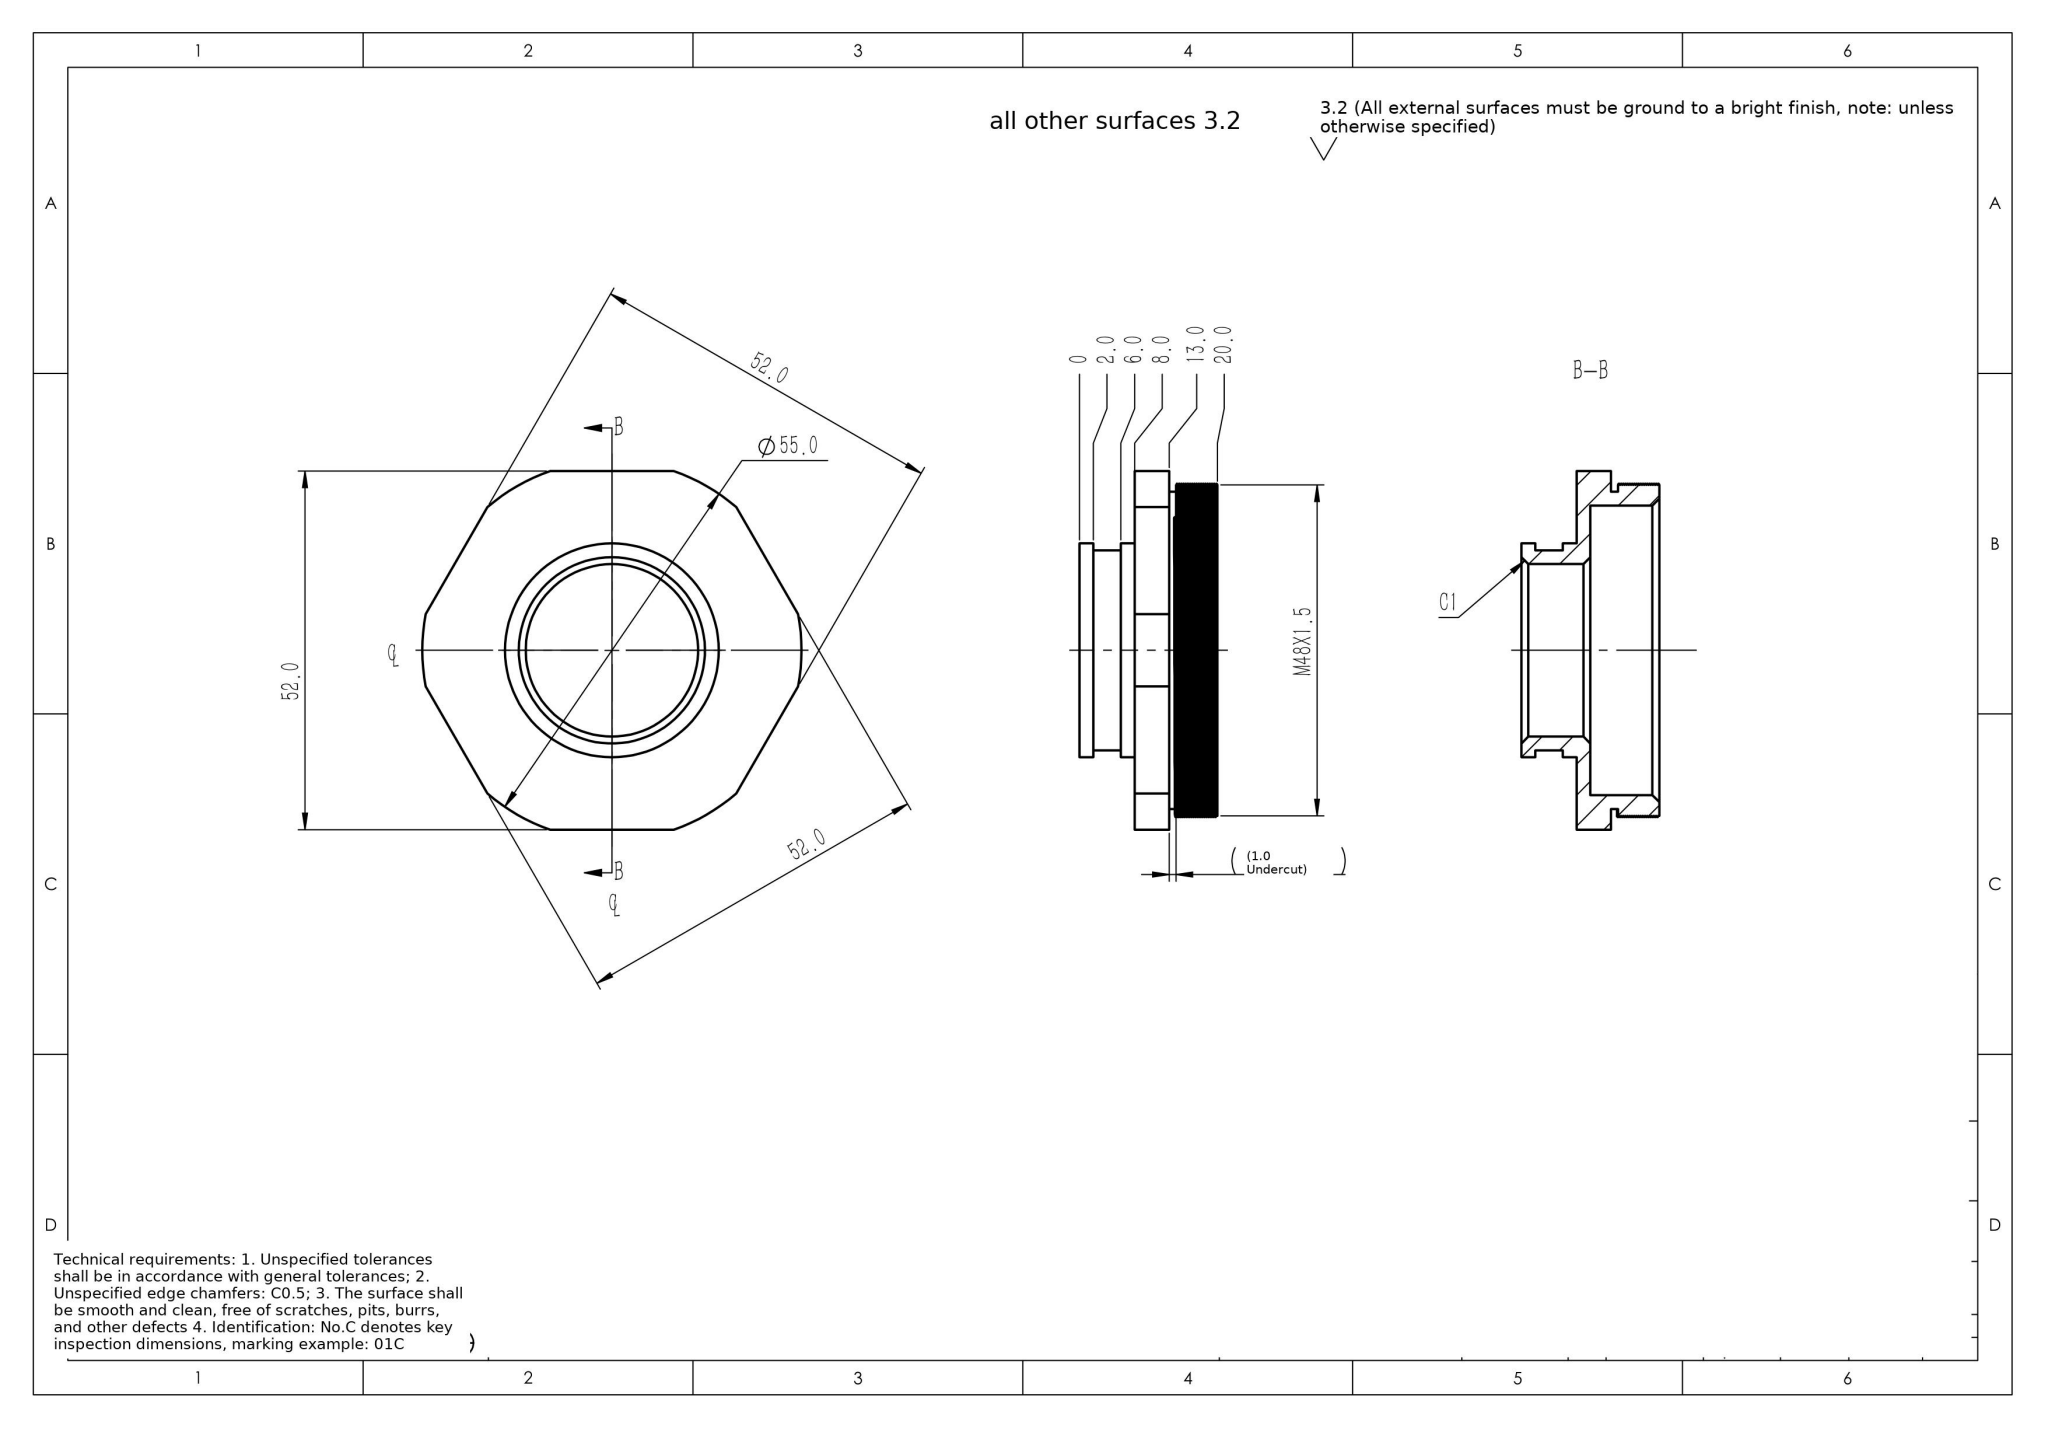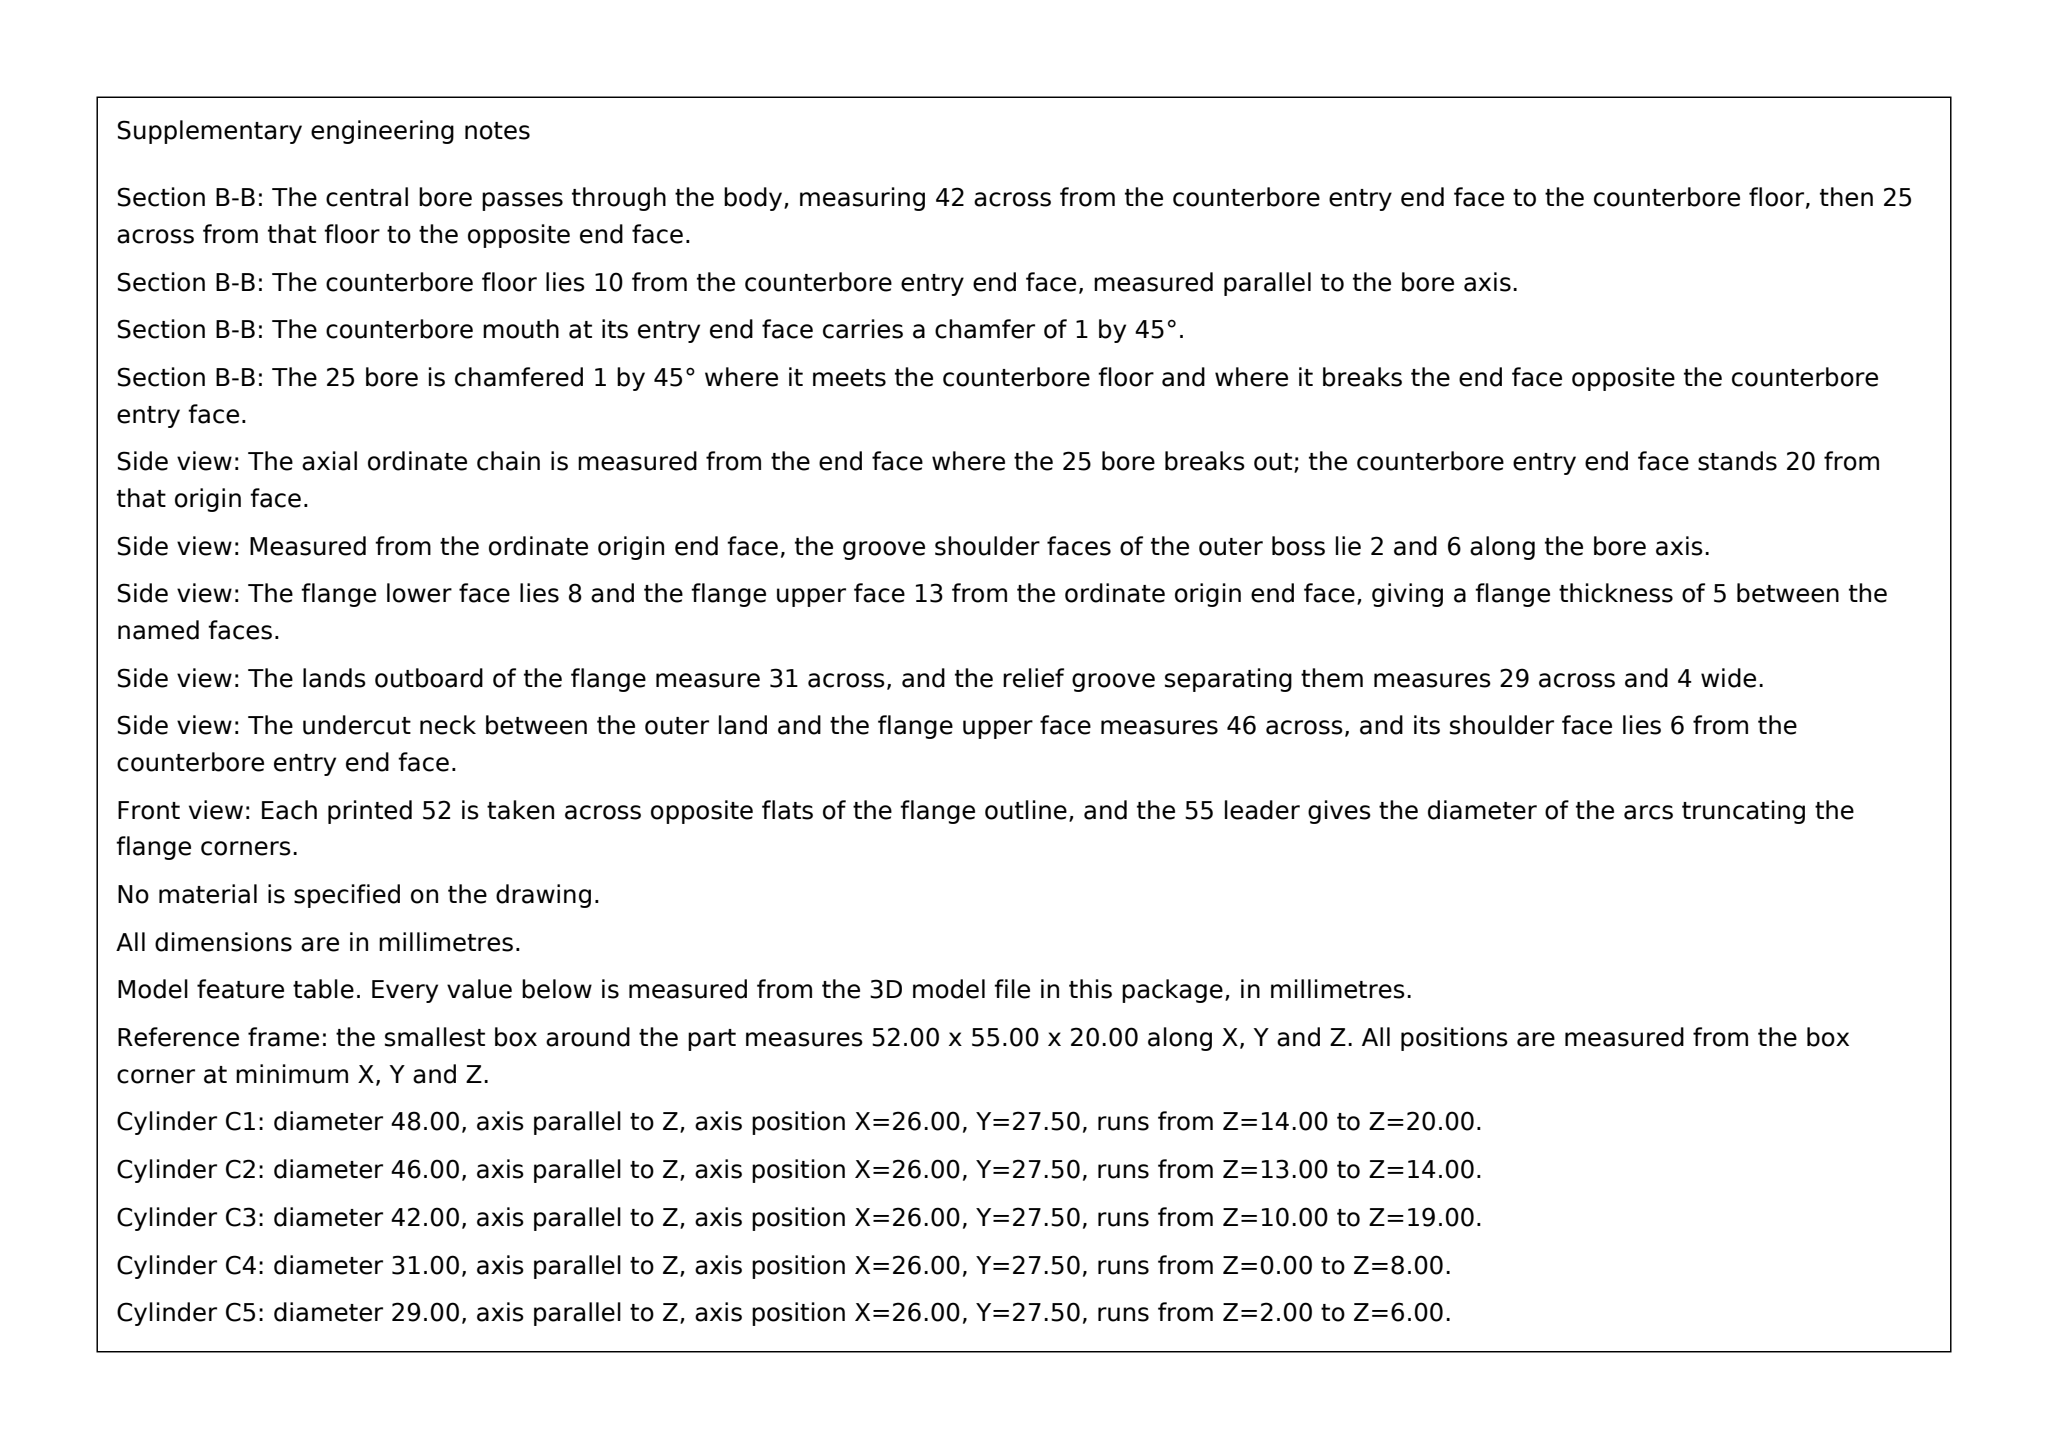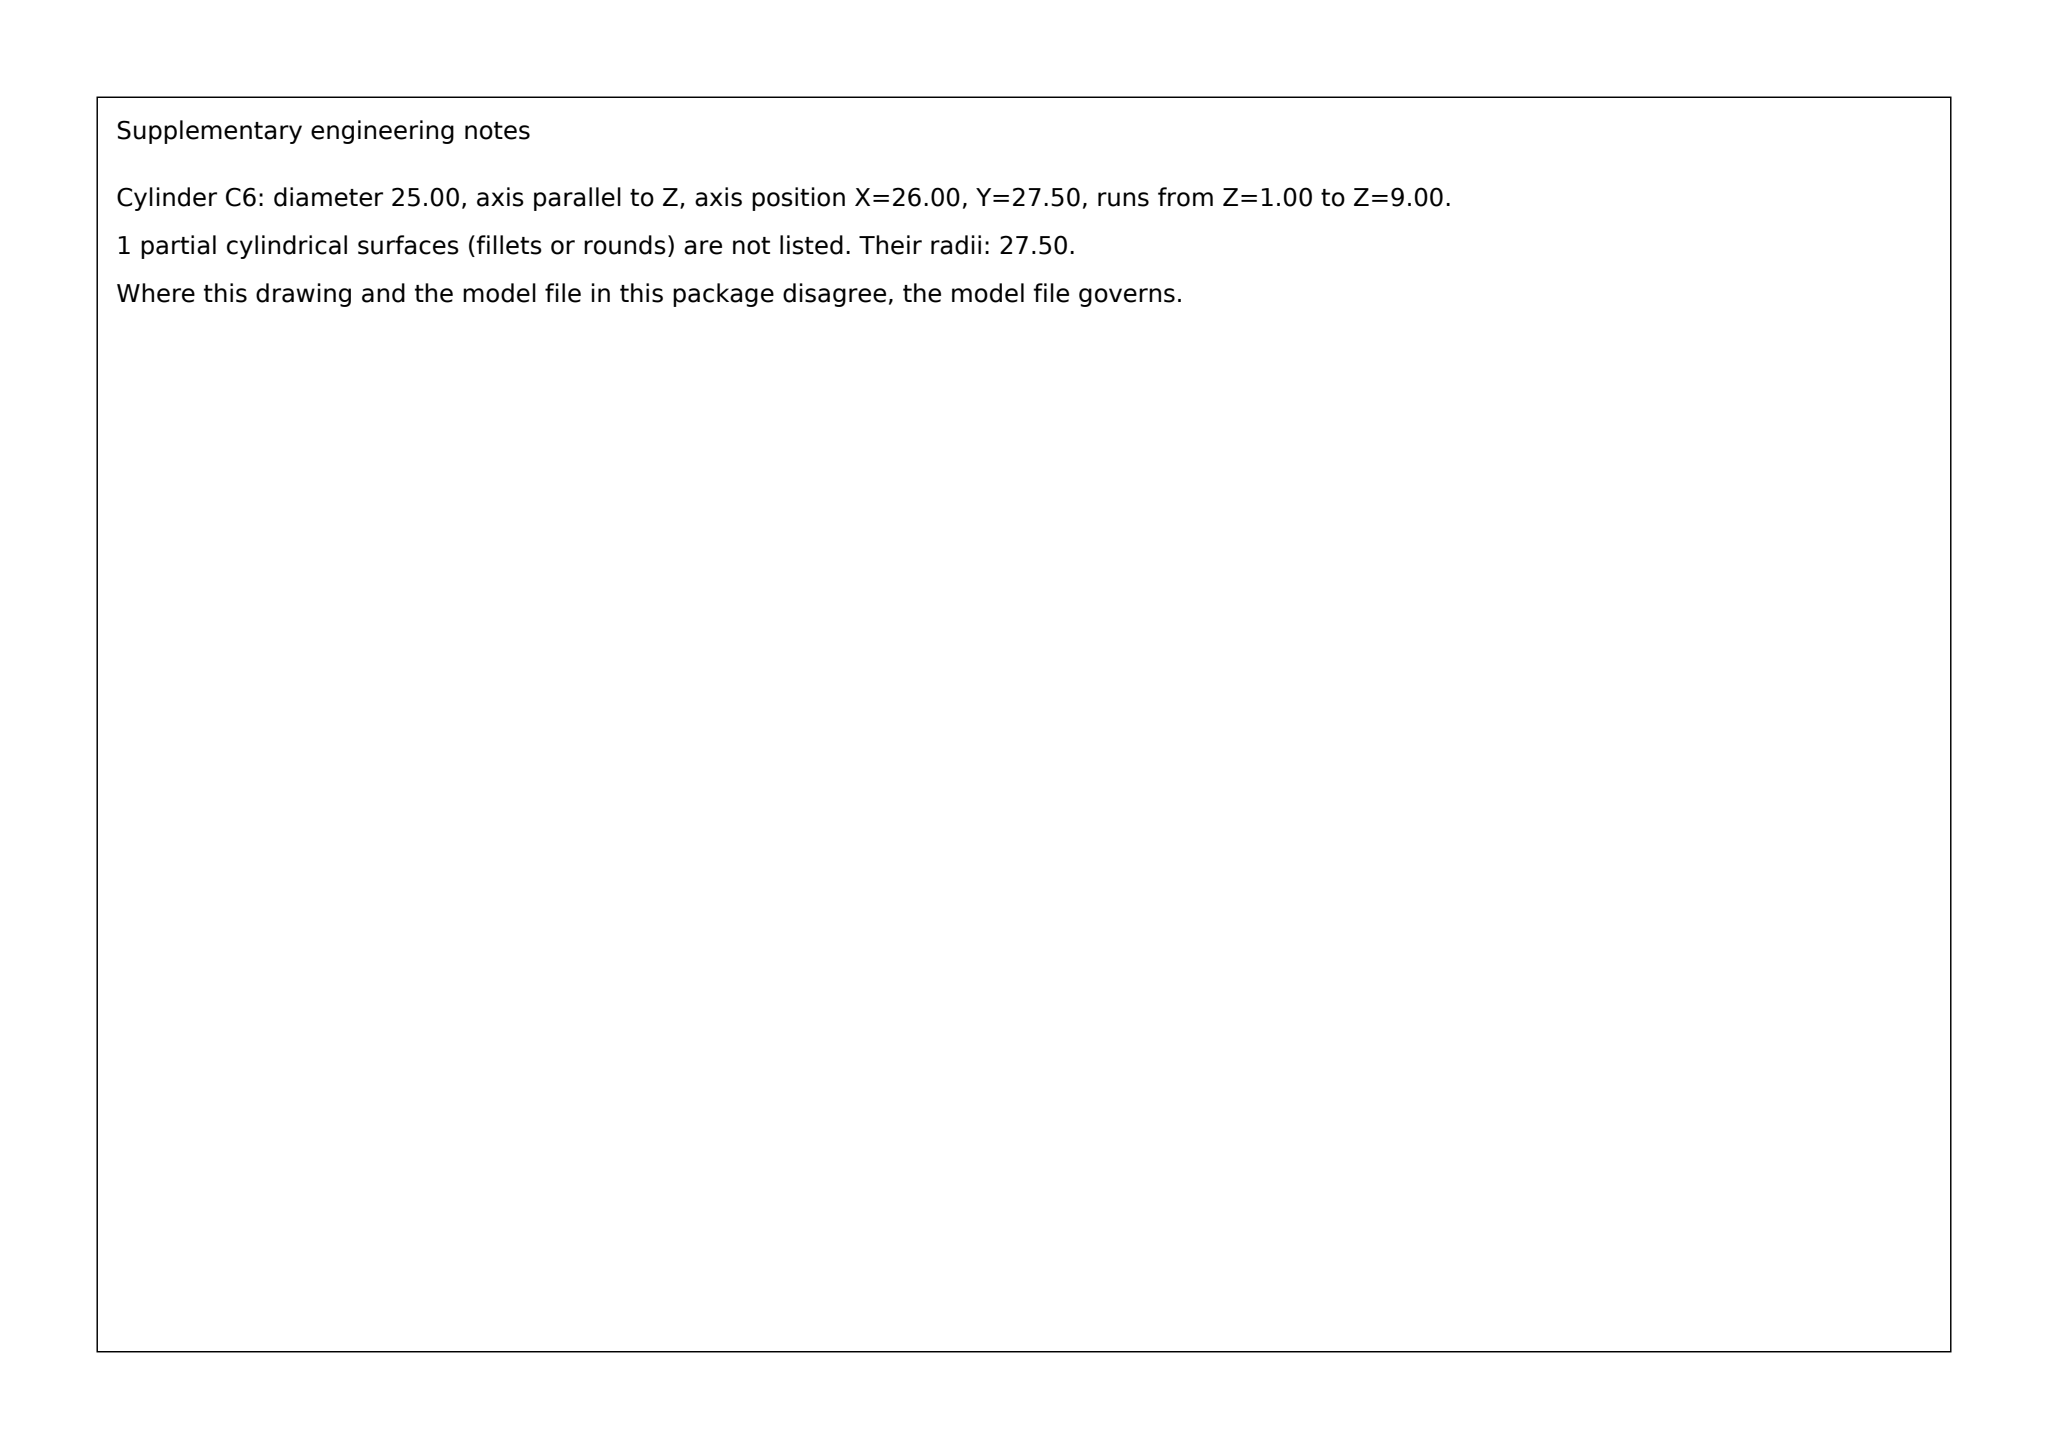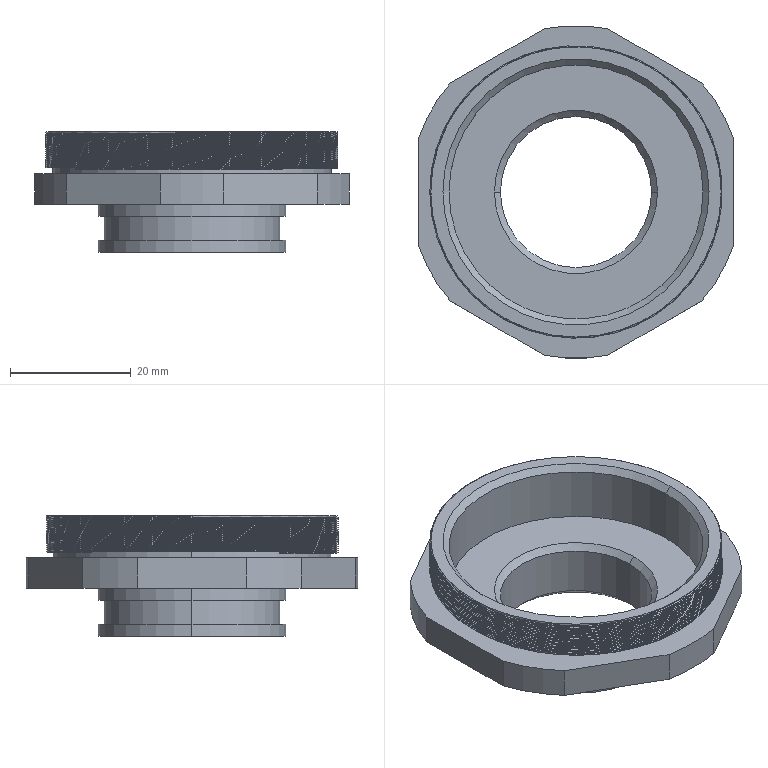Part | SolidWorks | mm | 1 solid | 83 faces | box 52 x 55 x 20 mm | volume 10695 mm3 | cylinder 57 | plane 16 | cone 6 | spline 4 | commonest cylinder face diameters 48 x39 55 x6 31 x4 42 x2 25 x2 29 x2 46 x2
Drawing notes:
Ø29 GROOVE DIA BETWEEN BOSSES, Z2-6 | from the solid: cylinder boss/shaft dia 29, z 2.0-6.0
CENTRAL THRU BORE Ø25, C1 AT Z0 END (90° x Ø27) | from the solid: hole/bore dia 25 z from 1.0 to 9.0; cone 90° ref dia 27 at z0-1
Ø25 BORE DP 10 FROM Z0 FACE; STEP UP TO Ø42 AT STA 10.0 | from the solid: Ø25 bore ends z=9.0 + 90° cone ref dia 25 z9-10; z-plane at 10.0
Ø42 C'BORE DP 10 FROM Z20 FACE, FLOOR AT STA 10.0 | from the solid: hole/bore dia 42 z from 10.0 to 19.0 + 90° cone ref dia 42 z19-20; z-plane 10.0 area 813
THD RELIEF GROOVE Ø46 x 1.0 WIDE, STA 13.0 TO 14.0 | from the solid: boss/shaft dia 46 z from 13.0 to 14.0